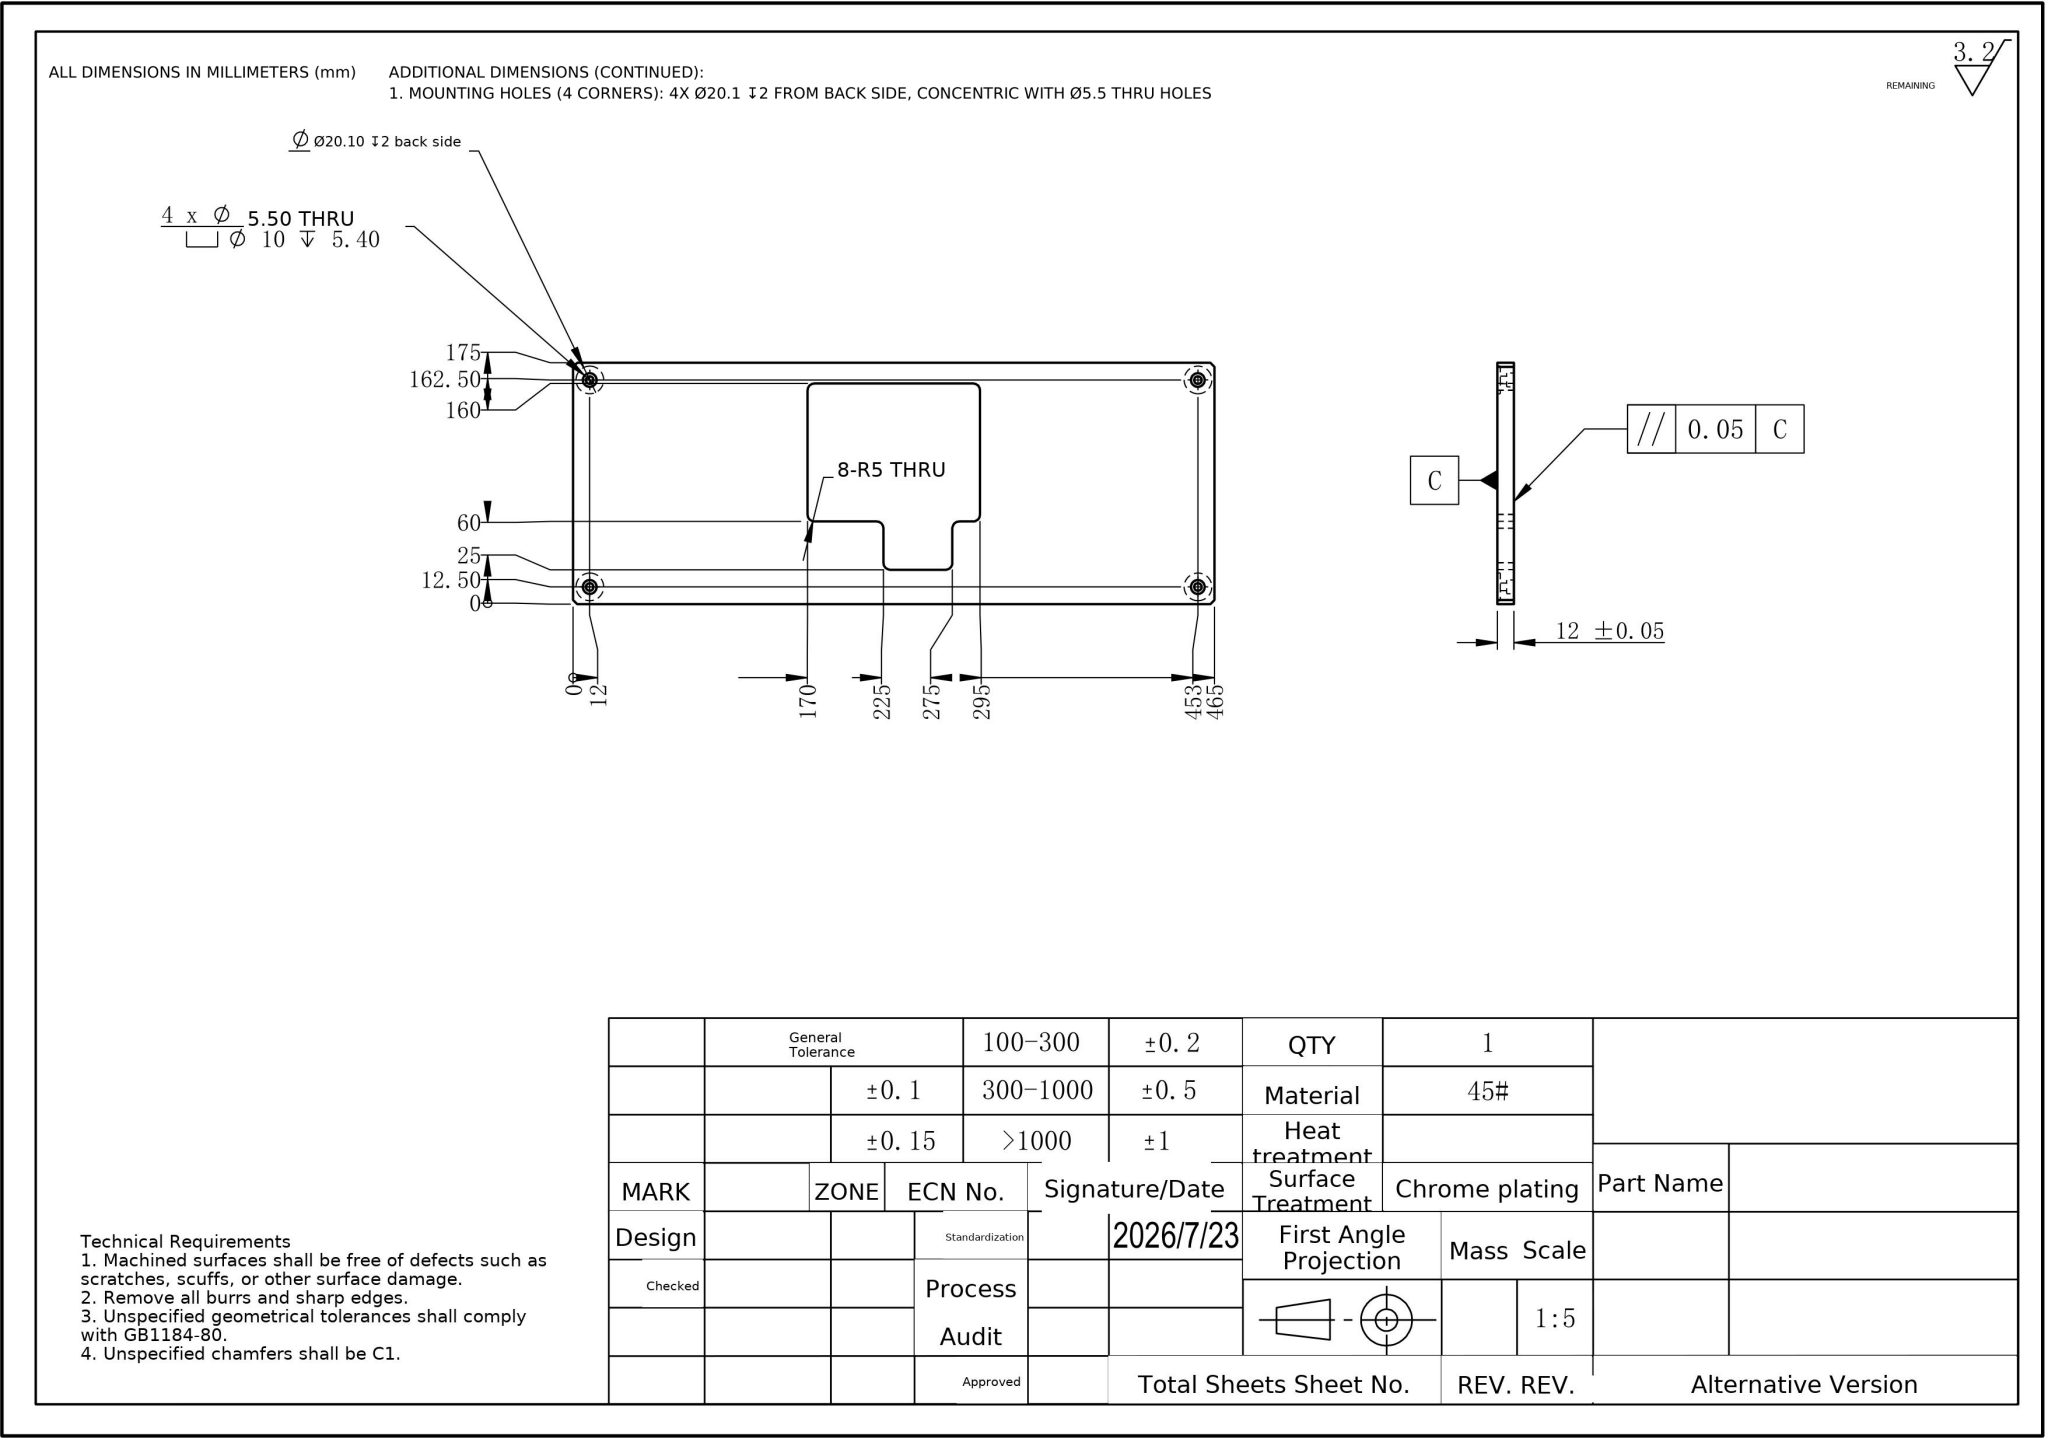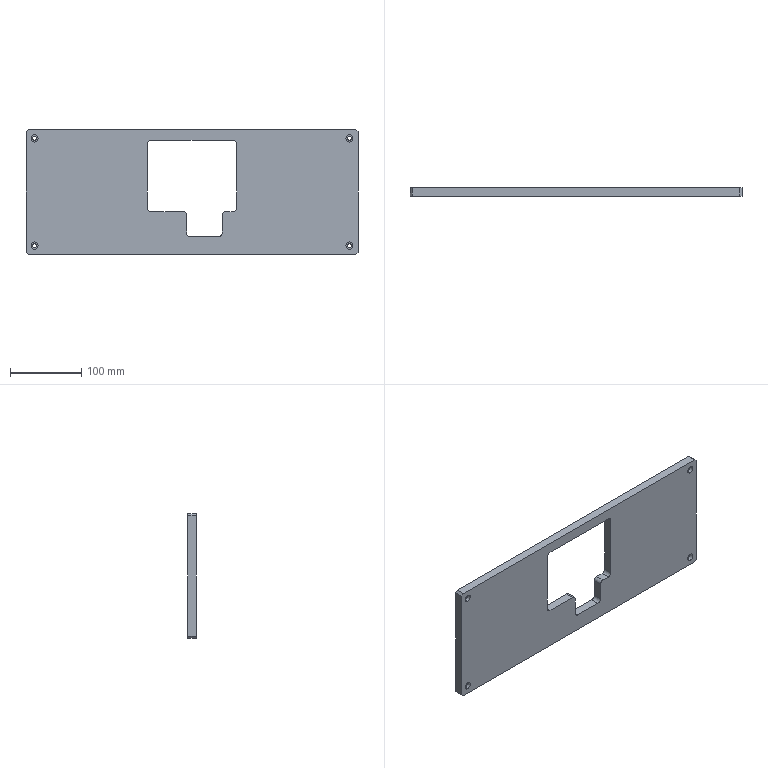Part | NX | mm | 1 solid | 58 faces | box 465 x 12 x 175 mm | volume 800869 mm3 | cylinder 32 | plane 26 | commonest cylinder face diameters 10 x16 5.5 x8 20.1 x8